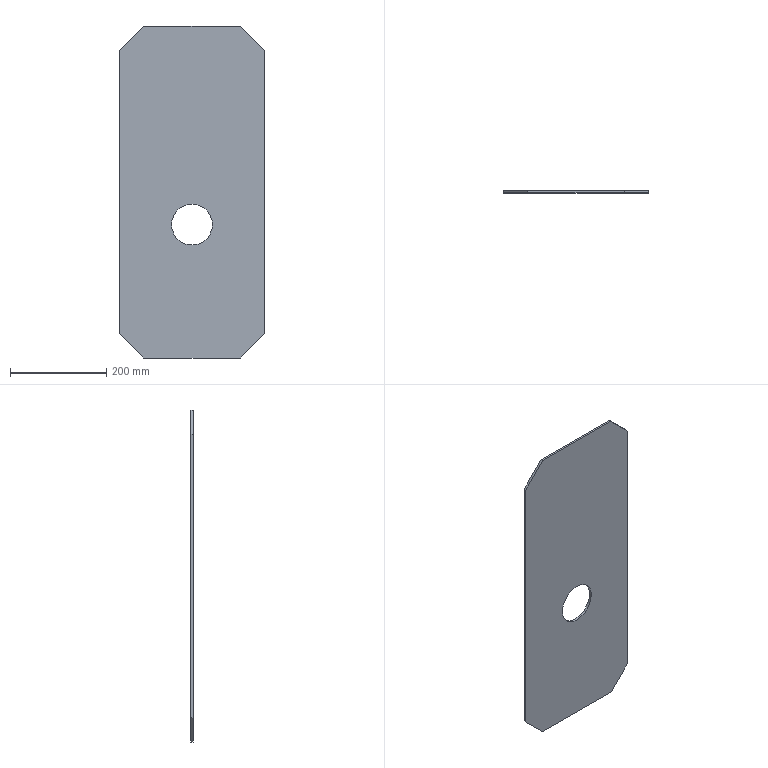Component | SolidWorks | LowerTensioningDeviceAssembly-1_ProtectivePlate-1 | 1 solid | 12 faces | box 300 x 5 x 690 mm | volume 981627 mm3 | plane 10 | cylinder 2 | commonest cylinder face diameters 85 x2
build123d program:
from build123d import *

# Parameters (mm, degrees)
SKETCH1_W           = 300
SKETCH1_H           = 690
BOSS_EXTRUDE1_DEPTH = 5
CHAMFER1_SIZE       = 50
SKETCH2_R           = 42.5
CUT_EXTRUDE1_DEPTH  = 20


with BuildPart() as part:
    # Sketch1 → Boss-Extrude1 (new body)
    with BuildSketch(Plane.XY):
        Rectangle(SKETCH1_W, SKETCH1_H)
    extrude(amount=BOSS_EXTRUDE1_DEPTH)

    # Chamfer1
    chamfer1_edges = [part.edges().sort_by_distance(p)[0] for p in [
        (150, -345, 2.5),
        (-150, -345, 2.5),
        (-150, 345, 2.5),
        (150, 345, 2.5),
    ]]
    chamfer(chamfer1_edges, length=CHAMFER1_SIZE)

    # Sketch2 → Cut-Extrude1 (cut)
    with BuildSketch(Plane.XY.offset(5)):
        with Locations((0, -67.8)):
            Circle(SKETCH2_R)
    extrude(amount=-CUT_EXTRUDE1_DEPTH, mode=Mode.SUBTRACT)


solid = part.part

# Placed as in the assembly
solid = solid.moved(Location((0, -275.1, 35), (90, 0, 0)))
STEP:
#1=COLOUR_RGB('',0.7922,0.8196,0.9333);
#2=FILL_AREA_STYLE_COLOUR('',#1);
#3=FILL_AREA_STYLE('',(#2));
#4=SURFACE_STYLE_FILL_AREA(#3);
#5=SURFACE_SIDE_STYLE('',(#4));
#6=SURFACE_STYLE_USAGE(.BOTH.,#5);
#7=PRESENTATION_STYLE_ASSIGNMENT((#6));
#8=CARTESIAN_POINT('',(1.673,-10.831,-1.291));
#9=VERTEX_POINT('',#8);
#10=CARTESIAN_POINT('',(-1.673,-10.831,-1.291));
#11=VERTEX_POINT('',#10);
#12=CARTESIAN_POINT('',(-0.,-10.831,-1.291));
#13=DIRECTION('',(0.,1.,0.));
#14=DIRECTION('',(-1.,0.,0.));
#15=AXIS2_PLACEMENT_3D('',#12,#13,#14);
#16=CIRCLE('',#15,1.673);
#17=EDGE_CURVE('',#9,#11,#16,.T.);
#18=ORIENTED_EDGE('',*,*,#17,.T.);
#19=CARTESIAN_POINT('',(-1.673,-11.028,-1.291));
#20=VERTEX_POINT('',#19);
#21=CARTESIAN_POINT('',(-1.673,-10.24,-1.291));
#22=DIRECTION('',(-0.,-1.,-0.));
#23=VECTOR('',#22,39.37);
#24=LINE('',#21,#23);
#25=EDGE_CURVE('',#11,#20,#24,.T.);
#26=ORIENTED_EDGE('',*,*,#25,.T.);
#27=CARTESIAN_POINT('',(1.673,-11.028,-1.291));
#28=VERTEX_POINT('',#27);
#29=CARTESIAN_POINT('',(-0.,-11.028,-1.291));
#30=DIRECTION('',(-0.,-1.,-0.));
#31=DIRECTION('',(1.,0.,-0.));
#32=AXIS2_PLACEMENT_3D('',#29,#30,#31);
#33=CIRCLE('',#32,1.673);
#34=EDGE_CURVE('',#20,#28,#33,.T.);
#35=ORIENTED_EDGE('',*,*,#34,.T.);
#36=CARTESIAN_POINT('',(1.673,-10.24,-1.291));
#37=DIRECTION('',(-0.,-1.,-0.));
#38=VECTOR('',#37,39.37);
#39=LINE('',#36,#38);
#40=EDGE_CURVE('',#9,#28,#39,.T.);
#41=ORIENTED_EDGE('',*,*,#40,.F.);
#42=EDGE_LOOP('',(#18,#26,#35,#41));
#43=FACE_OUTER_BOUND('',#42,.T.);
#44=CARTESIAN_POINT('',(-0.,-10.24,-1.291));
#45=DIRECTION('',(-0.,-1.,-0.));
#46=DIRECTION('',(1.,0.,-0.));
#47=AXIS2_PLACEMENT_3D('',#44,#45,#46);
#48=CYLINDRICAL_SURFACE('',#47,1.673);
#49=ADVANCED_FACE('',(#43),#48,.F.);
#50=CARTESIAN_POINT('',(5.906,-11.028,-10.236));
#51=VERTEX_POINT('',#50);
#52=CARTESIAN_POINT('',(5.906,-11.028,12.992));
#53=VERTEX_POINT('',#52);
#54=CARTESIAN_POINT('',(5.906,-11.028,-12.205));
#55=DIRECTION('',(0.,-0.,1.));
#56=VECTOR('',#55,39.37);
#57=LINE('',#54,#56);
#58=EDGE_CURVE('',#51,#53,#57,.T.);
#59=ORIENTED_EDGE('',*,*,#58,.F.);
#60=CARTESIAN_POINT('',(5.906,-10.831,-10.236));
#61=VERTEX_POINT('',#60);
#62=CARTESIAN_POINT('',(5.906,-11.028,-10.236));
#63=DIRECTION('',(0.,1.,0.));
#64=VECTOR('',#63,39.37);
#65=LINE('',#62,#64);
#66=EDGE_CURVE('',#51,#61,#65,.T.);
#67=ORIENTED_EDGE('',*,*,#66,.T.);
#68=CARTESIAN_POINT('',(5.906,-10.831,12.992));
#69=VERTEX_POINT('',#68);
#70=CARTESIAN_POINT('',(5.906,-10.831,-12.205));
#71=DIRECTION('',(0.,-0.,1.));
#72=VECTOR('',#71,39.37);
#73=LINE('',#70,#72);
#74=EDGE_CURVE('',#61,#69,#73,.T.);
#75=ORIENTED_EDGE('',*,*,#74,.T.);
#76=CARTESIAN_POINT('',(5.906,-11.028,12.992));
#77=DIRECTION('',(-0.,-1.,-0.));
#78=VECTOR('',#77,39.37);
#79=LINE('',#76,#78);
#80=EDGE_CURVE('',#69,#53,#79,.T.);
#81=ORIENTED_EDGE('',*,*,#80,.T.);
#82=EDGE_LOOP('',(#59,#67,#75,#81));
#83=FACE_OUTER_BOUND('',#82,.T.);
#84=CARTESIAN_POINT('',(5.906,-11.028,-12.205));
#85=DIRECTION('',(-1.,0.,0.));
#86=DIRECTION('',(-0.,-1.,-0.));
#87=AXIS2_PLACEMENT_3D('',#84,#85,#86);
#88=PLANE('',#87);
#89=ADVANCED_FACE('',(#83),#88,.F.);
#90=CARTESIAN_POINT('',(3.937,-10.831,14.961));
#91=VERTEX_POINT('',#90);
#92=CARTESIAN_POINT('',(-3.937,-10.831,14.961));
#93=VERTEX_POINT('',#92);
#94=CARTESIAN_POINT('',(-5.906,-10.831,14.961));
#95=DIRECTION('',(-1.,0.,0.));
#96=VECTOR('',#95,39.37);
#97=LINE('',#94,#96);
#98=EDGE_CURVE('',#91,#93,#97,.T.);
#99=ORIENTED_EDGE('',*,*,#98,.T.);
#100=CARTESIAN_POINT('',(-3.937,-11.028,14.961));
#101=VERTEX_POINT('',#100);
#102=CARTESIAN_POINT('',(-3.937,-11.028,14.961));
#103=DIRECTION('',(-0.,-1.,-0.));
#104=VECTOR('',#103,39.37);
#105=LINE('',#102,#104);
#106=EDGE_CURVE('',#93,#101,#105,.T.);
#107=ORIENTED_EDGE('',*,*,#106,.T.);
#108=CARTESIAN_POINT('',(3.937,-11.028,14.961));
#109=VERTEX_POINT('',#108);
#110=CARTESIAN_POINT('',(-5.906,-11.028,14.961));
#111=DIRECTION('',(-1.,0.,0.));
#112=VECTOR('',#111,39.37);
#113=LINE('',#110,#112);
#114=EDGE_CURVE('',#109,#101,#113,.T.);
#115=ORIENTED_EDGE('',*,*,#114,.F.);
#116=CARTESIAN_POINT('',(3.937,-11.028,14.961));
#117=DIRECTION('',(0.,1.,0.));
#118=VECTOR('',#117,39.37);
#119=LINE('',#116,#118);
#120=EDGE_CURVE('',#109,#91,#119,.T.);
#121=ORIENTED_EDGE('',*,*,#120,.T.);
#122=EDGE_LOOP('',(#99,#107,#115,#121));
#123=FACE_OUTER_BOUND('',#122,.T.);
#124=CARTESIAN_POINT('',(-5.906,-11.028,14.961));
#125=DIRECTION('',(-0.,0.,-1.));
#126=DIRECTION('',(0.,1.,0.));
#127=AXIS2_PLACEMENT_3D('',#124,#125,#126);
#128=PLANE('',#127);
#129=ADVANCED_FACE('',(#123),#128,.F.);
#130=CARTESIAN_POINT('',(-5.906,-10.831,12.992));
#131=VERTEX_POINT('',#130);
#132=CARTESIAN_POINT('',(-5.906,-10.831,-10.236));
#133=VERTEX_POINT('',#132);
#134=CARTESIAN_POINT('',(-5.906,-10.831,-12.205));
#135=DIRECTION('',(-0.,0.,-1.));
#136=VECTOR('',#135,39.37);
#137=LINE('',#134,#136);
#138=EDGE_CURVE('',#131,#133,#137,.T.);
#139=ORIENTED_EDGE('',*,*,#138,.T.);
#140=CARTESIAN_POINT('',(-5.906,-11.028,-10.236));
#141=VERTEX_POINT('',#140);
#142=CARTESIAN_POINT('',(-5.906,-11.028,-10.236));
#143=DIRECTION('',(-0.,-1.,-0.));
#144=VECTOR('',#143,39.37);
#145=LINE('',#142,#144);
#146=EDGE_CURVE('',#133,#141,#145,.T.);
#147=ORIENTED_EDGE('',*,*,#146,.T.);
#148=CARTESIAN_POINT('',(-5.906,-11.028,12.992));
#149=VERTEX_POINT('',#148);
#150=CARTESIAN_POINT('',(-5.906,-11.028,-12.205));
#151=DIRECTION('',(-0.,0.,-1.));
#152=VECTOR('',#151,39.37);
#153=LINE('',#150,#152);
#154=EDGE_CURVE('',#149,#141,#153,.T.);
#155=ORIENTED_EDGE('',*,*,#154,.F.);
#156=CARTESIAN_POINT('',(-5.906,-11.028,12.992));
#157=DIRECTION('',(0.,1.,0.));
#158=VECTOR('',#157,39.37);
#159=LINE('',#156,#158);
#160=EDGE_CURVE('',#149,#131,#159,.T.);
#161=ORIENTED_EDGE('',*,*,#160,.T.);
#162=EDGE_LOOP('',(#139,#147,#155,#161));
#163=FACE_OUTER_BOUND('',#162,.T.);
#164=CARTESIAN_POINT('',(-5.906,-11.028,-12.205));
#165=DIRECTION('',(1.,-0.,-0.));
#166=DIRECTION('',(0.,1.,0.));
#167=AXIS2_PLACEMENT_3D('',#164,#165,#166);
#168=PLANE('',#167);
#169=ADVANCED_FACE('',(#163),#168,.F.);
#170=CARTESIAN_POINT('',(-3.937,-11.028,-12.205));
#171=VERTEX_POINT('',#170);
#172=CARTESIAN_POINT('',(3.937,-11.028,-12.205));
#173=VERTEX_POINT('',#172);
#174=CARTESIAN_POINT('',(-5.906,-11.028,-12.205));
#175=DIRECTION('',(1.,-0.,-0.));
#176=VECTOR('',#175,39.37);
#177=LINE('',#174,#176);
#178=EDGE_CURVE('',#171,#173,#177,.T.);
#179=ORIENTED_EDGE('',*,*,#178,.F.);
#180=CARTESIAN_POINT('',(-3.937,-10.831,-12.205));
#181=VERTEX_POINT('',#180);
#182=CARTESIAN_POINT('',(-3.937,-11.028,-12.205));
#183=DIRECTION('',(0.,1.,0.));
#184=VECTOR('',#183,39.37);
#185=LINE('',#182,#184);
#186=EDGE_CURVE('',#171,#181,#185,.T.);
#187=ORIENTED_EDGE('',*,*,#186,.T.);
#188=CARTESIAN_POINT('',(3.937,-10.831,-12.205));
#189=VERTEX_POINT('',#188);
#190=CARTESIAN_POINT('',(-5.906,-10.831,-12.205));
#191=DIRECTION('',(1.,-0.,-0.));
#192=VECTOR('',#191,39.37);
#193=LINE('',#190,#192);
#194=EDGE_CURVE('',#181,#189,#193,.T.);
#195=ORIENTED_EDGE('',*,*,#194,.T.);
#196=CARTESIAN_POINT('',(3.937,-11.028,-12.205));
#197=DIRECTION('',(-0.,-1.,-0.));
#198=VECTOR('',#197,39.37);
#199=LINE('',#196,#198);
#200=EDGE_CURVE('',#189,#173,#199,.T.);
#201=ORIENTED_EDGE('',*,*,#200,.T.);
#202=EDGE_LOOP('',(#179,#187,#195,#201));
#203=FACE_OUTER_BOUND('',#202,.T.);
#204=CARTESIAN_POINT('',(-5.906,-11.028,-12.205));
#205=DIRECTION('',(0.,-0.,1.));
#206=DIRECTION('',(-0.,-1.,-0.));
#207=AXIS2_PLACEMENT_3D('',#204,#205,#206);
#208=PLANE('',#207);
#209=ADVANCED_FACE('',(#203),#208,.F.);
#210=CARTESIAN_POINT('',(-0.,-11.028,-1.291));
#211=DIRECTION('',(-0.,-1.,-0.));
#212=DIRECTION('',(1.,0.,-0.));
#213=AXIS2_PLACEMENT_3D('',#210,#211,#212);
#214=CIRCLE('',#213,1.673);
#215=EDGE_CURVE('',#28,#20,#214,.T.);
#216=ORIENTED_EDGE('',*,*,#215,.F.);
#217=ORIENTED_EDGE('',*,*,#34,.F.);
#218=EDGE_LOOP('',(#216,#217));
#219=FACE_BOUND('',#218,.T.);
#220=ORIENTED_EDGE('',*,*,#154,.T.);
#221=CARTESIAN_POINT('',(-3.937,-11.028,-12.205));
#222=DIRECTION('',(0.7071,0.,-0.7071));
#223=VECTOR('',#222,39.37);
#224=LINE('',#221,#223);
#225=EDGE_CURVE('',#141,#171,#224,.T.);
#226=ORIENTED_EDGE('',*,*,#225,.T.);
#227=ORIENTED_EDGE('',*,*,#178,.T.);
#228=CARTESIAN_POINT('',(5.906,-11.028,-10.236));
#229=DIRECTION('',(0.7071,-0.,0.7071));
#230=VECTOR('',#229,39.37);
#231=LINE('',#228,#230);
#232=EDGE_CURVE('',#173,#51,#231,.T.);
#233=ORIENTED_EDGE('',*,*,#232,.T.);
#234=ORIENTED_EDGE('',*,*,#58,.T.);
#235=CARTESIAN_POINT('',(3.937,-11.028,14.961));
#236=DIRECTION('',(-0.7071,-0.,0.7071));
#237=VECTOR('',#236,39.37);
#238=LINE('',#235,#237);
#239=EDGE_CURVE('',#53,#109,#238,.T.);
#240=ORIENTED_EDGE('',*,*,#239,.T.);
#241=ORIENTED_EDGE('',*,*,#114,.T.);
#242=CARTESIAN_POINT('',(-5.906,-11.028,12.992));
#243=DIRECTION('',(-0.7071,0.,-0.7071));
#244=VECTOR('',#243,39.37);
#245=LINE('',#242,#244);
#246=EDGE_CURVE('',#101,#149,#245,.T.);
#247=ORIENTED_EDGE('',*,*,#246,.T.);
#248=EDGE_LOOP('',(#220,#226,#227,#233,#234,#240,#241,#247));
#249=FACE_OUTER_BOUND('',#248,.T.);
#250=CARTESIAN_POINT('',(-0.,-11.028,1.378));
#251=DIRECTION('',(0.,1.,0.));
#252=DIRECTION('',(-1.,0.,0.));
#253=AXIS2_PLACEMENT_3D('',#250,#251,#252);
#254=PLANE('',#253);
#255=ADVANCED_FACE('',(#219,#249),#254,.F.);
#256=ORIENTED_EDGE('',*,*,#17,.F.);
#257=CARTESIAN_POINT('',(-0.,-10.831,-1.291));
#258=DIRECTION('',(0.,1.,0.));
#259=DIRECTION('',(-1.,0.,0.));
#260=AXIS2_PLACEMENT_3D('',#257,#258,#259);
#261=CIRCLE('',#260,1.673);
#262=EDGE_CURVE('',#11,#9,#261,.T.);
#263=ORIENTED_EDGE('',*,*,#262,.F.);
#264=EDGE_LOOP('',(#256,#263));
#265=FACE_BOUND('',#264,.T.);
#266=ORIENTED_EDGE('',*,*,#194,.F.);
#267=CARTESIAN_POINT('',(-8.76,-10.831,-7.382));
#268=DIRECTION('',(-0.7071,-0.,0.7071));
#269=VECTOR('',#268,39.37);
#270=LINE('',#267,#269);
#271=EDGE_CURVE('',#181,#133,#270,.T.);
#272=ORIENTED_EDGE('',*,*,#271,.T.);
#273=ORIENTED_EDGE('',*,*,#138,.F.);
#274=CARTESIAN_POINT('',(-8.76,-10.831,10.138));
#275=DIRECTION('',(0.7071,-0.,0.7071));
#276=VECTOR('',#275,39.37);
#277=LINE('',#274,#276);
#278=EDGE_CURVE('',#131,#93,#277,.T.);
#279=ORIENTED_EDGE('',*,*,#278,.T.);
#280=ORIENTED_EDGE('',*,*,#98,.F.);
#281=CARTESIAN_POINT('',(8.76,-10.831,10.138));
#282=DIRECTION('',(0.7071,0.,-0.7071));
#283=VECTOR('',#282,39.37);
#284=LINE('',#281,#283);
#285=EDGE_CURVE('',#91,#69,#284,.T.);
#286=ORIENTED_EDGE('',*,*,#285,.T.);
#287=ORIENTED_EDGE('',*,*,#74,.F.);
#288=CARTESIAN_POINT('',(8.76,-10.831,-7.382));
#289=DIRECTION('',(-0.7071,0.,-0.7071));
#290=VECTOR('',#289,39.37);
#291=LINE('',#288,#290);
#292=EDGE_CURVE('',#61,#189,#291,.T.);
#293=ORIENTED_EDGE('',*,*,#292,.T.);
#294=EDGE_LOOP('',(#266,#272,#273,#279,#280,#286,#287,#293));
#295=FACE_OUTER_BOUND('',#294,.T.);
#296=CARTESIAN_POINT('',(-0.,-10.831,1.378));
#297=DIRECTION('',(0.,1.,0.));
#298=DIRECTION('',(-1.,0.,0.));
#299=AXIS2_PLACEMENT_3D('',#296,#297,#298);
#300=PLANE('',#299);
#301=ADVANCED_FACE('',(#265,#295),#300,.T.);
#302=ORIENTED_EDGE('',*,*,#225,.F.);
#303=ORIENTED_EDGE('',*,*,#146,.F.);
#304=ORIENTED_EDGE('',*,*,#271,.F.);
#305=ORIENTED_EDGE('',*,*,#186,.F.);
#306=EDGE_LOOP('',(#302,#303,#304,#305));
#307=FACE_OUTER_BOUND('',#306,.T.);
#308=CARTESIAN_POINT('',(-3.937,-11.028,-12.205));
#309=DIRECTION('',(0.7071,-0.,0.7071));
#310=DIRECTION('',(0.,1.,0.));
#311=AXIS2_PLACEMENT_3D('',#308,#309,#310);
#312=PLANE('',#311);
#313=ADVANCED_FACE('',(#307),#312,.F.);
#314=ORIENTED_EDGE('',*,*,#232,.F.);
#315=ORIENTED_EDGE('',*,*,#200,.F.);
#316=ORIENTED_EDGE('',*,*,#292,.F.);
#317=ORIENTED_EDGE('',*,*,#66,.F.);
#318=EDGE_LOOP('',(#314,#315,#316,#317));
#319=FACE_OUTER_BOUND('',#318,.T.);
#320=CARTESIAN_POINT('',(5.906,-11.028,-10.236));
#321=DIRECTION('',(-0.7071,-0.,0.7071));
#322=DIRECTION('',(0.,1.,0.));
#323=AXIS2_PLACEMENT_3D('',#320,#321,#322);
#324=PLANE('',#323);
#325=ADVANCED_FACE('',(#319),#324,.F.);
#326=ORIENTED_EDGE('',*,*,#246,.F.);
#327=ORIENTED_EDGE('',*,*,#106,.F.);
#328=ORIENTED_EDGE('',*,*,#278,.F.);
#329=ORIENTED_EDGE('',*,*,#160,.F.);
#330=EDGE_LOOP('',(#326,#327,#328,#329));
#331=FACE_OUTER_BOUND('',#330,.T.);
#332=CARTESIAN_POINT('',(-5.906,-11.028,12.992));
#333=DIRECTION('',(0.7071,0.,-0.7071));
#334=DIRECTION('',(0.,1.,0.));
#335=AXIS2_PLACEMENT_3D('',#332,#333,#334);
#336=PLANE('',#335);
#337=ADVANCED_FACE('',(#331),#336,.F.);
#338=ORIENTED_EDGE('',*,*,#239,.F.);
#339=ORIENTED_EDGE('',*,*,#80,.F.);
#340=ORIENTED_EDGE('',*,*,#285,.F.);
#341=ORIENTED_EDGE('',*,*,#120,.F.);
#342=EDGE_LOOP('',(#338,#339,#340,#341));
#343=FACE_OUTER_BOUND('',#342,.T.);
#344=CARTESIAN_POINT('',(3.937,-11.028,14.961));
#345=DIRECTION('',(-0.7071,0.,-0.7071));
#346=DIRECTION('',(0.,1.,0.));
#347=AXIS2_PLACEMENT_3D('',#344,#345,#346);
#348=PLANE('',#347);
#349=ADVANCED_FACE('',(#343),#348,.F.);
#350=ORIENTED_EDGE('',*,*,#25,.F.);
#351=ORIENTED_EDGE('',*,*,#262,.T.);
#352=ORIENTED_EDGE('',*,*,#40,.T.);
#353=ORIENTED_EDGE('',*,*,#215,.T.);
#354=EDGE_LOOP('',(#350,#351,#352,#353));
#355=FACE_OUTER_BOUND('',#354,.T.);
#356=CARTESIAN_POINT('',(-0.,-10.24,-1.291));
#357=DIRECTION('',(-0.,-1.,-0.));
#358=DIRECTION('',(1.,0.,-0.));
#359=AXIS2_PLACEMENT_3D('',#356,#357,#358);
#360=CYLINDRICAL_SURFACE('',#359,1.673);
#361=ADVANCED_FACE('',(#355),#360,.F.);
#362=CLOSED_SHELL('',(#49,#89,#129,#169,#209,#255,#301,#313,#325,#337,#349,#361));
#363=MANIFOLD_SOLID_BREP('',#362);
#364=STYLED_ITEM('',(#7),#363);
#365=PRESENTATION_LAYER_ASSIGNMENT('','',(#364));
#366=(LENGTH_UNIT()NAMED_UNIT(*)SI_UNIT($,.METRE.));
#367=LENGTH_MEASURE_WITH_UNIT(LENGTH_MEASURE(0.0254),#366);
#368=DIMENSIONAL_EXPONENTS(1.,0.,0.,0.,0.,0.,0.);
#369=(CONVERSION_BASED_UNIT('',#367)LENGTH_UNIT()NAMED_UNIT(#368));
#370=UNCERTAINTY_MEASURE_WITH_UNIT(LENGTH_MEASURE(0.00001),#369,'','');
#371=(NAMED_UNIT(*)PLANE_ANGLE_UNIT()SI_UNIT($,.RADIAN.));
#372=(NAMED_UNIT(*)SI_UNIT($,.STERADIAN.)SOLID_ANGLE_UNIT());
#373=(GEOMETRIC_REPRESENTATION_CONTEXT(3)GLOBAL_UNCERTAINTY_ASSIGNED_CONTEXT((#370))GLOBAL_UNIT_ASSIGNED_CONTEXT((#369,#371,#372))REPRESENTATION_CONTEXT('',''));
#374=MECHANICAL_DESIGN_GEOMETRIC_PRESENTATION_REPRESENTATION('',(#364),#373);
#375=CARTESIAN_POINT('',(0.,0.,0.));
#376=DIRECTION('',(0.,0.,1.));
#377=DIRECTION('',(1.,0.,0.));
#378=AXIS2_PLACEMENT_3D('',#375,#376,#377);
#379=(LENGTH_UNIT()NAMED_UNIT(*)SI_UNIT($,.METRE.));
#380=LENGTH_MEASURE_WITH_UNIT(LENGTH_MEASURE(0.0254),#379);
#381=DIMENSIONAL_EXPONENTS(1.,0.,0.,0.,0.,0.,0.);
#382=(CONVERSION_BASED_UNIT('',#380)LENGTH_UNIT()NAMED_UNIT(#381));
#383=UNCERTAINTY_MEASURE_WITH_UNIT(LENGTH_MEASURE(0.00001),#382,'','');
#384=(NAMED_UNIT(*)PLANE_ANGLE_UNIT()SI_UNIT($,.RADIAN.));
#385=(NAMED_UNIT(*)SI_UNIT($,.STERADIAN.)SOLID_ANGLE_UNIT());
#386=(GEOMETRIC_REPRESENTATION_CONTEXT(3)GLOBAL_UNCERTAINTY_ASSIGNED_CONTEXT((#383))GLOBAL_UNIT_ASSIGNED_CONTEXT((#382,#384,#385))REPRESENTATION_CONTEXT('',''));
#387=ADVANCED_BREP_SHAPE_REPRESENTATION('',(#363,#378),#386);